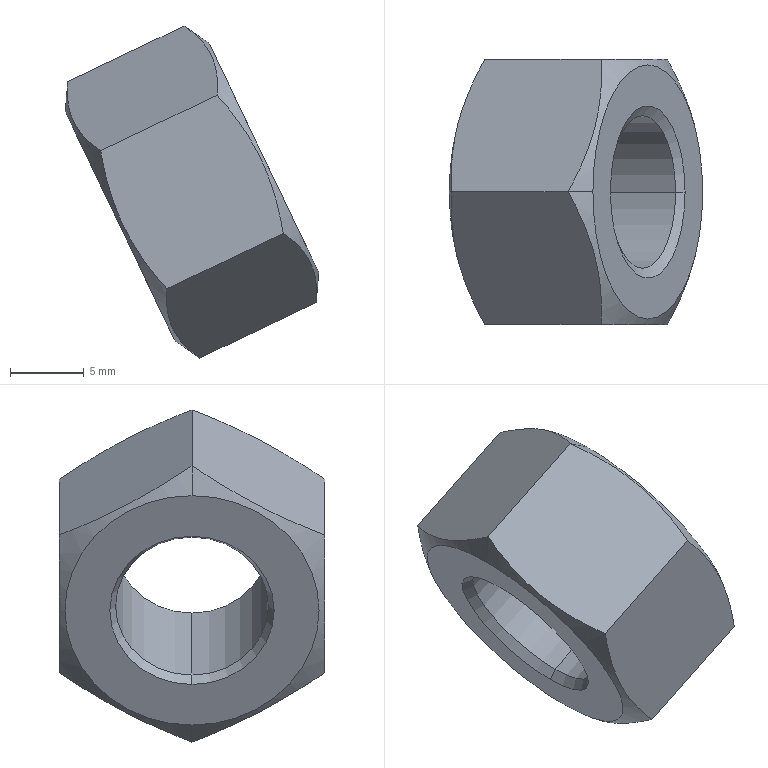Component | SolidWorks | hex nuts 1-fine pitch-grades ab gb-1 | 1 solid | 18 faces | box 17.19 x 18 x 22.53 mm | volume 2080 mm3 | cone 8 | plane 8 | cylinder 2 | commonest cylinder face diameters 10.376 x2
STEP:
#1=COLOUR_RGB('',0.7922,0.8196,0.9333);
#2=FILL_AREA_STYLE_COLOUR('',#1);
#3=FILL_AREA_STYLE('',(#2));
#4=SURFACE_STYLE_FILL_AREA(#3);
#5=SURFACE_SIDE_STYLE('',(#4));
#6=SURFACE_STYLE_USAGE(.BOTH.,#5);
#7=PRESENTATION_STYLE_ASSIGNMENT((#6));
#8=CARTESIAN_POINT('',(1.881,9.843,19.173));
#9=VERTEX_POINT('',#8);
#10=CARTESIAN_POINT('',(2.058,9.843,18.805));
#11=VERTEX_POINT('',#10);
#12=CARTESIAN_POINT('',(1.97,9.843,18.989));
#13=DIRECTION('',(0.902,-0.,0.4318));
#14=DIRECTION('',(-0.4318,-0.,0.902));
#15=AXIS2_PLACEMENT_3D('',#12,#13,#14);
#16=CIRCLE('',#15,0.2043);
#17=EDGE_CURVE('',#9,#11,#16,.T.);
#18=ORIENTED_EDGE('',*,*,#17,.F.);
#19=CARTESIAN_POINT('',(1.884,9.843,19.204));
#20=VERTEX_POINT('',#19);
#21=CARTESIAN_POINT('',(1.881,9.843,19.173));
#22=DIRECTION('',(0.07705,-0.,0.997));
#23=VECTOR('',#22,39.37);
#24=LINE('',#21,#23);
#25=EDGE_CURVE('',#9,#20,#24,.T.);
#26=ORIENTED_EDGE('',*,*,#25,.T.);
#27=CARTESIAN_POINT('',(2.083,9.843,18.788));
#28=VERTEX_POINT('',#27);
#29=CARTESIAN_POINT('',(1.983,9.843,18.996));
#30=DIRECTION('',(-0.902,0.,-0.4318));
#31=DIRECTION('',(-0.4318,-0.,0.902));
#32=AXIS2_PLACEMENT_3D('',#29,#30,#31);
#33=CIRCLE('',#32,0.2308);
#34=EDGE_CURVE('',#28,#20,#33,.T.);
#35=ORIENTED_EDGE('',*,*,#34,.F.);
#36=CARTESIAN_POINT('',(2.058,9.843,18.805));
#37=DIRECTION('',(0.8249,0.,-0.5652));
#38=VECTOR('',#37,39.37);
#39=LINE('',#36,#38);
#40=EDGE_CURVE('',#11,#28,#39,.T.);
#41=ORIENTED_EDGE('',*,*,#40,.F.);
#42=EDGE_LOOP('',(#18,#26,#35,#41));
#43=FACE_OUTER_BOUND('',#42,.T.);
#44=CARTESIAN_POINT('',(1.97,9.843,18.989));
#45=DIRECTION('',(0.902,-0.,0.4318));
#46=DIRECTION('',(0.4318,0.,-0.902));
#47=AXIS2_PLACEMENT_3D('',#44,#45,#46);
#48=CONICAL_SURFACE('',#47,0.2043,1.047);
#49=ADVANCED_FACE('',(#43),#48,.F.);
#50=CARTESIAN_POINT('',(1.712,9.843,18.64));
#51=VERTEX_POINT('',#50);
#52=CARTESIAN_POINT('',(1.536,9.843,19.008));
#53=VERTEX_POINT('',#52);
#54=CARTESIAN_POINT('',(1.624,9.843,18.824));
#55=DIRECTION('',(-0.902,0.,-0.4318));
#56=DIRECTION('',(-0.4318,-0.,0.902));
#57=AXIS2_PLACEMENT_3D('',#54,#55,#56);
#58=CIRCLE('',#57,0.2043);
#59=EDGE_CURVE('',#51,#53,#58,.T.);
#60=ORIENTED_EDGE('',*,*,#59,.F.);
#61=CARTESIAN_POINT('',(1.695,9.843,18.614));
#62=VERTEX_POINT('',#61);
#63=CARTESIAN_POINT('',(1.695,9.843,18.614));
#64=DIRECTION('',(-0.5652,0.,-0.8249));
#65=VECTOR('',#64,39.37);
#66=LINE('',#63,#65);
#67=EDGE_CURVE('',#51,#62,#66,.T.);
#68=ORIENTED_EDGE('',*,*,#67,.T.);
#69=CARTESIAN_POINT('',(1.505,9.843,19.01));
#70=VERTEX_POINT('',#69);
#71=CARTESIAN_POINT('',(1.6,9.843,18.812));
#72=DIRECTION('',(0.902,-0.,0.4318));
#73=DIRECTION('',(-0.4318,-0.,0.902));
#74=AXIS2_PLACEMENT_3D('',#71,#72,#73);
#75=CIRCLE('',#74,0.2196);
#76=EDGE_CURVE('',#70,#62,#75,.T.);
#77=ORIENTED_EDGE('',*,*,#76,.F.);
#78=CARTESIAN_POINT('',(1.505,9.843,19.01));
#79=DIRECTION('',(-0.997,-0.,0.07705));
#80=VECTOR('',#79,39.37);
#81=LINE('',#78,#80);
#82=EDGE_CURVE('',#53,#70,#81,.T.);
#83=ORIENTED_EDGE('',*,*,#82,.F.);
#84=EDGE_LOOP('',(#60,#68,#77,#83));
#85=FACE_OUTER_BOUND('',#84,.T.);
#86=CARTESIAN_POINT('',(1.6,9.843,18.812));
#87=DIRECTION('',(-0.902,0.,-0.4318));
#88=DIRECTION('',(-0.4318,-0.,0.902));
#89=AXIS2_PLACEMENT_3D('',#86,#87,#88);
#90=CONICAL_SURFACE('',#89,0.2196,0.5236);
#91=ADVANCED_FACE('',(#85),#90,.F.);
#92=CARTESIAN_POINT('',(1.837,9.843,19.302));
#93=VERTEX_POINT('',#92);
#94=CARTESIAN_POINT('',(2.13,9.843,18.69));
#95=VERTEX_POINT('',#94);
#96=CARTESIAN_POINT('',(1.983,9.843,18.996));
#97=DIRECTION('',(-0.902,0.,-0.4318));
#98=DIRECTION('',(-0.4318,-0.,0.902));
#99=AXIS2_PLACEMENT_3D('',#96,#97,#98);
#100=CIRCLE('',#99,0.3396);
#101=EDGE_CURVE('',#93,#95,#100,.T.);
#102=ORIENTED_EDGE('',*,*,#101,.T.);
#103=CARTESIAN_POINT('',(2.124,9.843,18.609));
#104=VERTEX_POINT('',#103);
#105=CARTESIAN_POINT('',(2.13,9.843,18.69));
#106=DIRECTION('',(-0.07705,0.,-0.997));
#107=VECTOR('',#106,39.37);
#108=LINE('',#105,#107);
#109=EDGE_CURVE('',#95,#104,#108,.T.);
#110=ORIENTED_EDGE('',*,*,#109,.T.);
#111=CARTESIAN_POINT('',(2.036,10.197,18.794));
#112=VERTEX_POINT('',#111);
#113=CARTESIAN_POINT('',(2.124,9.843,18.609));
#114=CARTESIAN_POINT('',(2.125,9.871,18.629));
#115=CARTESIAN_POINT('',(2.125,9.901,18.647));
#116=CARTESIAN_POINT('',(2.121,9.959,18.683));
#117=CARTESIAN_POINT('',(2.116,9.989,18.7));
#118=CARTESIAN_POINT('',(2.105,10.034,18.723));
#119=CARTESIAN_POINT('',(2.1,10.05,18.731));
#120=CARTESIAN_POINT('',(2.09,10.079,18.745));
#121=CARTESIAN_POINT('',(2.084,10.094,18.752));
#122=CARTESIAN_POINT('',(2.066,10.139,18.771));
#123=CARTESIAN_POINT('',(2.051,10.168,18.783));
#124=CARTESIAN_POINT('',(2.036,10.197,18.794));
#125=B_SPLINE_CURVE_WITH_KNOTS('',3,(#113,#114,#115,#116,#117,#118,#119,#120,#121,#122,#123,#124),.UNSPECIFIED.,.F.,.F.,(4,2,2,2,2,4),(0.00000024,0.002624,0.005248,0.00656,0.007872,0.0105),.UNSPECIFIED.);
#126=EDGE_CURVE('',#104,#112,#125,.T.);
#127=ORIENTED_EDGE('',*,*,#126,.T.);
#128=CARTESIAN_POINT('',(1.859,10.197,19.163));
#129=VERTEX_POINT('',#128);
#130=CARTESIAN_POINT('',(2.036,10.197,18.794));
#131=CARTESIAN_POINT('',(2.03,10.197,18.828));
#132=CARTESIAN_POINT('',(2.023,10.197,18.862));
#133=CARTESIAN_POINT('',(2.008,10.197,18.911));
#134=CARTESIAN_POINT('',(2.002,10.197,18.928));
#135=CARTESIAN_POINT('',(1.99,10.197,18.961));
#136=CARTESIAN_POINT('',(1.983,10.197,18.977));
#137=CARTESIAN_POINT('',(1.961,10.197,19.023));
#138=CARTESIAN_POINT('',(1.943,10.197,19.053));
#139=CARTESIAN_POINT('',(1.904,10.197,19.11));
#140=CARTESIAN_POINT('',(1.882,10.197,19.137));
#141=CARTESIAN_POINT('',(1.859,10.197,19.163));
#142=B_SPLINE_CURVE_WITH_KNOTS('',3,(#130,#131,#132,#133,#134,#135,#136,#137,#138,#139,#140,#141),.UNSPECIFIED.,.F.,.F.,(4,2,2,2,2,4),(0.003845,0.006467,0.007778,0.009089,0.01171,0.01433),.UNSPECIFIED.);
#143=EDGE_CURVE('',#112,#129,#142,.T.);
#144=ORIENTED_EDGE('',*,*,#143,.T.);
#145=CARTESIAN_POINT('',(1.771,9.843,19.348));
#146=VERTEX_POINT('',#145);
#147=CARTESIAN_POINT('',(1.859,10.197,19.163));
#148=CARTESIAN_POINT('',(1.86,10.168,19.182));
#149=CARTESIAN_POINT('',(1.86,10.139,19.201));
#150=CARTESIAN_POINT('',(1.856,10.08,19.236));
#151=CARTESIAN_POINT('',(1.851,10.05,19.253));
#152=CARTESIAN_POINT('',(1.84,10.005,19.277));
#153=CARTESIAN_POINT('',(1.835,9.99,19.284));
#154=CARTESIAN_POINT('',(1.825,9.96,19.299));
#155=CARTESIAN_POINT('',(1.819,9.945,19.305));
#156=CARTESIAN_POINT('',(1.801,9.901,19.325));
#157=CARTESIAN_POINT('',(1.786,9.871,19.337));
#158=CARTESIAN_POINT('',(1.771,9.843,19.348));
#159=B_SPLINE_CURVE_WITH_KNOTS('',3,(#147,#148,#149,#150,#151,#152,#153,#154,#155,#156,#157,#158),.UNSPECIFIED.,.F.,.F.,(4,2,2,2,2,4),(0.00000024,0.002624,0.005248,0.00656,0.007872,0.0105),.UNSPECIFIED.);
#160=EDGE_CURVE('',#129,#146,#159,.T.);
#161=ORIENTED_EDGE('',*,*,#160,.T.);
#162=CARTESIAN_POINT('',(1.837,9.843,19.302));
#163=DIRECTION('',(-0.8249,-0.,0.5652));
#164=VECTOR('',#163,39.37);
#165=LINE('',#162,#164);
#166=EDGE_CURVE('',#93,#146,#165,.T.);
#167=ORIENTED_EDGE('',*,*,#166,.F.);
#168=EDGE_LOOP('',(#102,#110,#127,#144,#161,#167));
#169=FACE_OUTER_BOUND('',#168,.T.);
#170=CARTESIAN_POINT('',(1.983,9.843,18.996));
#171=DIRECTION('',(-0.902,0.,-0.4318));
#172=DIRECTION('',(-0.4318,-0.,0.902));
#173=AXIS2_PLACEMENT_3D('',#170,#171,#172);
#174=CONICAL_SURFACE('',#173,0.3396,1.047);
#175=ADVANCED_FACE('',(#169),#174,.T.);
#176=CARTESIAN_POINT('',(1.453,9.843,19.119));
#177=VERTEX_POINT('',#176);
#178=CARTESIAN_POINT('',(1.747,9.843,18.506));
#179=VERTEX_POINT('',#178);
#180=CARTESIAN_POINT('',(1.6,9.843,18.812));
#181=DIRECTION('',(-0.902,0.,-0.4318));
#182=DIRECTION('',(-0.4318,-0.,0.902));
#183=AXIS2_PLACEMENT_3D('',#180,#181,#182);
#184=CIRCLE('',#183,0.3396);
#185=EDGE_CURVE('',#177,#179,#184,.T.);
#186=ORIENTED_EDGE('',*,*,#185,.F.);
#187=CARTESIAN_POINT('',(1.459,9.843,19.199));
#188=VERTEX_POINT('',#187);
#189=CARTESIAN_POINT('',(1.459,9.843,19.199));
#190=DIRECTION('',(0.07705,-0.,0.997));
#191=VECTOR('',#190,39.37);
#192=LINE('',#189,#191);
#193=EDGE_CURVE('',#177,#188,#192,.T.);
#194=ORIENTED_EDGE('',*,*,#193,.T.);
#195=CARTESIAN_POINT('',(1.548,10.197,19.014));
#196=VERTEX_POINT('',#195);
#197=CARTESIAN_POINT('',(1.459,9.843,19.199));
#198=CARTESIAN_POINT('',(1.458,9.871,19.179));
#199=CARTESIAN_POINT('',(1.458,9.901,19.161));
#200=CARTESIAN_POINT('',(1.463,9.959,19.125));
#201=CARTESIAN_POINT('',(1.468,9.989,19.109));
#202=CARTESIAN_POINT('',(1.479,10.034,19.085));
#203=CARTESIAN_POINT('',(1.483,10.05,19.078));
#204=CARTESIAN_POINT('',(1.493,10.079,19.063));
#205=CARTESIAN_POINT('',(1.499,10.094,19.056));
#206=CARTESIAN_POINT('',(1.517,10.139,19.037));
#207=CARTESIAN_POINT('',(1.532,10.168,19.025));
#208=CARTESIAN_POINT('',(1.548,10.197,19.014));
#209=B_SPLINE_CURVE_WITH_KNOTS('',3,(#197,#198,#199,#200,#201,#202,#203,#204,#205,#206,#207,#208),.UNSPECIFIED.,.F.,.F.,(4,2,2,2,2,4),(0.00000024,0.002624,0.005248,0.00656,0.007872,0.0105),.UNSPECIFIED.);
#210=EDGE_CURVE('',#188,#196,#209,.T.);
#211=ORIENTED_EDGE('',*,*,#210,.T.);
#212=CARTESIAN_POINT('',(1.724,10.197,18.645));
#213=VERTEX_POINT('',#212);
#214=CARTESIAN_POINT('',(1.548,10.197,19.014));
#215=CARTESIAN_POINT('',(1.554,10.197,18.98));
#216=CARTESIAN_POINT('',(1.561,10.197,18.946));
#217=CARTESIAN_POINT('',(1.581,10.197,18.879));
#218=CARTESIAN_POINT('',(1.593,10.197,18.847));
#219=CARTESIAN_POINT('',(1.615,10.197,18.8));
#220=CARTESIAN_POINT('',(1.623,10.197,18.785));
#221=CARTESIAN_POINT('',(1.641,10.197,18.755));
#222=CARTESIAN_POINT('',(1.65,10.197,18.74));
#223=CARTESIAN_POINT('',(1.68,10.197,18.698));
#224=CARTESIAN_POINT('',(1.702,10.197,18.671));
#225=CARTESIAN_POINT('',(1.724,10.197,18.645));
#226=B_SPLINE_CURVE_WITH_KNOTS('',3,(#214,#215,#216,#217,#218,#219,#220,#221,#222,#223,#224,#225),.UNSPECIFIED.,.F.,.F.,(4,2,2,2,2,4),(0.009237,0.01187,0.0145,0.01581,0.01712,0.01975),.UNSPECIFIED.);
#227=EDGE_CURVE('',#196,#213,#226,.T.);
#228=ORIENTED_EDGE('',*,*,#227,.T.);
#229=CARTESIAN_POINT('',(1.813,9.843,18.461));
#230=VERTEX_POINT('',#229);
#231=CARTESIAN_POINT('',(1.724,10.197,18.645));
#232=CARTESIAN_POINT('',(1.723,10.168,18.626));
#233=CARTESIAN_POINT('',(1.723,10.139,18.607));
#234=CARTESIAN_POINT('',(1.728,10.08,18.572));
#235=CARTESIAN_POINT('',(1.733,10.05,18.555));
#236=CARTESIAN_POINT('',(1.744,10.005,18.532));
#237=CARTESIAN_POINT('',(1.748,9.99,18.524));
#238=CARTESIAN_POINT('',(1.758,9.96,18.51));
#239=CARTESIAN_POINT('',(1.764,9.945,18.503));
#240=CARTESIAN_POINT('',(1.782,9.901,18.483));
#241=CARTESIAN_POINT('',(1.797,9.871,18.472));
#242=CARTESIAN_POINT('',(1.813,9.843,18.461));
#243=B_SPLINE_CURVE_WITH_KNOTS('',3,(#231,#232,#233,#234,#235,#236,#237,#238,#239,#240,#241,#242),.UNSPECIFIED.,.F.,.F.,(4,2,2,2,2,4),(0.00000024,0.002624,0.005248,0.00656,0.007872,0.0105),.UNSPECIFIED.);
#244=EDGE_CURVE('',#213,#230,#243,.T.);
#245=ORIENTED_EDGE('',*,*,#244,.T.);
#246=CARTESIAN_POINT('',(1.813,9.843,18.461));
#247=DIRECTION('',(0.8249,0.,-0.5652));
#248=VECTOR('',#247,39.37);
#249=LINE('',#246,#248);
#250=EDGE_CURVE('',#179,#230,#249,.T.);
#251=ORIENTED_EDGE('',*,*,#250,.F.);
#252=EDGE_LOOP('',(#186,#194,#211,#228,#245,#251));
#253=FACE_OUTER_BOUND('',#252,.T.);
#254=CARTESIAN_POINT('',(1.636,9.843,18.83));
#255=DIRECTION('',(0.902,-0.,0.4318));
#256=DIRECTION('',(0.4318,0.,-0.902));
#257=AXIS2_PLACEMENT_3D('',#254,#255,#256);
#258=CONICAL_SURFACE('',#257,0.4091,1.047);
#259=ADVANCED_FACE('',(#253),#258,.T.);
#260=ORIENTED_EDGE('',*,*,#59,.T.);
#261=CARTESIAN_POINT('',(1.512,9.843,18.997));
#262=DIRECTION('',(0.902,-0.,0.4318));
#263=VECTOR('',#262,39.37);
#264=LINE('',#261,#263);
#265=EDGE_CURVE('',#53,#9,#264,.T.);
#266=ORIENTED_EDGE('',*,*,#265,.T.);
#267=ORIENTED_EDGE('',*,*,#17,.T.);
#268=CARTESIAN_POINT('',(1.688,9.843,18.628));
#269=DIRECTION('',(0.902,-0.,0.4318));
#270=VECTOR('',#269,39.37);
#271=LINE('',#268,#270);
#272=EDGE_CURVE('',#51,#11,#271,.T.);
#273=ORIENTED_EDGE('',*,*,#272,.F.);
#274=EDGE_LOOP('',(#260,#266,#267,#273));
#275=FACE_OUTER_BOUND('',#274,.T.);
#276=CARTESIAN_POINT('',(1.6,9.843,18.812));
#277=DIRECTION('',(0.902,-0.,0.4318));
#278=DIRECTION('',(0.4318,0.,-0.902));
#279=AXIS2_PLACEMENT_3D('',#276,#277,#278);
#280=CYLINDRICAL_SURFACE('',#279,0.2043);
#281=ADVANCED_FACE('',(#275),#280,.F.);
#282=CARTESIAN_POINT('',(1.859,9.488,19.163));
#283=VERTEX_POINT('',#282);
#284=CARTESIAN_POINT('',(2.036,9.488,18.794));
#285=VERTEX_POINT('',#284);
#286=CARTESIAN_POINT('',(1.859,9.488,19.163));
#287=CARTESIAN_POINT('',(1.882,9.488,19.137));
#288=CARTESIAN_POINT('',(1.904,9.488,19.11));
#289=CARTESIAN_POINT('',(1.943,9.488,19.053));
#290=CARTESIAN_POINT('',(1.961,9.488,19.023));
#291=CARTESIAN_POINT('',(1.983,9.488,18.977));
#292=CARTESIAN_POINT('',(1.99,9.488,18.961));
#293=CARTESIAN_POINT('',(2.002,9.488,18.928));
#294=CARTESIAN_POINT('',(2.008,9.488,18.911));
#295=CARTESIAN_POINT('',(2.023,9.488,18.862));
#296=CARTESIAN_POINT('',(2.03,9.488,18.828));
#297=CARTESIAN_POINT('',(2.036,9.488,18.794));
#298=B_SPLINE_CURVE_WITH_KNOTS('',3,(#286,#287,#288,#289,#290,#291,#292,#293,#294,#295,#296,#297),.UNSPECIFIED.,.F.,.F.,(4,2,2,2,2,4),(0.009237,0.01187,0.0145,0.01581,0.01712,0.01975),.UNSPECIFIED.);
#299=EDGE_CURVE('',#283,#285,#298,.T.);
#300=ORIENTED_EDGE('',*,*,#299,.F.);
#301=CARTESIAN_POINT('',(1.548,9.488,19.014));
#302=VERTEX_POINT('',#301);
#303=CARTESIAN_POINT('',(1.512,9.488,18.997));
#304=DIRECTION('',(0.902,-0.,0.4318));
#305=VECTOR('',#304,39.37);
#306=LINE('',#303,#305);
#307=EDGE_CURVE('',#302,#283,#306,.T.);
#308=ORIENTED_EDGE('',*,*,#307,.F.);
#309=CARTESIAN_POINT('',(1.724,9.488,18.645));
#310=VERTEX_POINT('',#309);
#311=CARTESIAN_POINT('',(1.724,9.488,18.645));
#312=CARTESIAN_POINT('',(1.702,9.488,18.671));
#313=CARTESIAN_POINT('',(1.68,9.488,18.698));
#314=CARTESIAN_POINT('',(1.65,9.488,18.74));
#315=CARTESIAN_POINT('',(1.641,9.488,18.755));
#316=CARTESIAN_POINT('',(1.623,9.488,18.785));
#317=CARTESIAN_POINT('',(1.615,9.488,18.8));
#318=CARTESIAN_POINT('',(1.593,9.488,18.847));
#319=CARTESIAN_POINT('',(1.581,9.488,18.879));
#320=CARTESIAN_POINT('',(1.561,9.488,18.946));
#321=CARTESIAN_POINT('',(1.554,9.488,18.98));
#322=CARTESIAN_POINT('',(1.548,9.488,19.014));
#323=B_SPLINE_CURVE_WITH_KNOTS('',3,(#311,#312,#313,#314,#315,#316,#317,#318,#319,#320,#321,#322),.UNSPECIFIED.,.F.,.F.,(4,2,2,2,2,4),(0.003845,0.006467,0.007778,0.009089,0.01171,0.01433),.UNSPECIFIED.);
#324=EDGE_CURVE('',#310,#302,#323,.T.);
#325=ORIENTED_EDGE('',*,*,#324,.F.);
#326=CARTESIAN_POINT('',(1.688,9.488,18.628));
#327=DIRECTION('',(0.902,-0.,0.4318));
#328=VECTOR('',#327,39.37);
#329=LINE('',#326,#328);
#330=EDGE_CURVE('',#310,#285,#329,.T.);
#331=ORIENTED_EDGE('',*,*,#330,.T.);
#332=EDGE_LOOP('',(#300,#308,#325,#331));
#333=FACE_OUTER_BOUND('',#332,.T.);
#334=CARTESIAN_POINT('',(1.512,9.488,18.997));
#335=DIRECTION('',(0.,-1.,-0.));
#336=DIRECTION('',(0.4318,0.,-0.902));
#337=AXIS2_PLACEMENT_3D('',#334,#335,#336);
#338=PLANE('',#337);
#339=ADVANCED_FACE('',(#333),#338,.T.);
#340=CARTESIAN_POINT('',(1.771,9.843,19.348));
#341=CARTESIAN_POINT('',(1.786,9.814,19.337));
#342=CARTESIAN_POINT('',(1.801,9.784,19.325));
#343=CARTESIAN_POINT('',(1.825,9.726,19.299));
#344=CARTESIAN_POINT('',(1.836,9.696,19.285));
#345=CARTESIAN_POINT('',(1.847,9.651,19.261));
#346=CARTESIAN_POINT('',(1.85,9.635,19.253));
#347=CARTESIAN_POINT('',(1.855,9.606,19.236));
#348=CARTESIAN_POINT('',(1.857,9.591,19.228));
#349=CARTESIAN_POINT('',(1.86,9.546,19.201));
#350=CARTESIAN_POINT('',(1.86,9.517,19.182));
#351=CARTESIAN_POINT('',(1.859,9.488,19.163));
#352=B_SPLINE_CURVE_WITH_KNOTS('',3,(#340,#341,#342,#343,#344,#345,#346,#347,#348,#349,#350,#351),.UNSPECIFIED.,.F.,.F.,(4,2,2,2,2,4),(0.00000024,0.002624,0.005248,0.00656,0.007872,0.0105),.UNSPECIFIED.);
#353=EDGE_CURVE('',#146,#283,#352,.T.);
#354=ORIENTED_EDGE('',*,*,#353,.F.);
#355=CARTESIAN_POINT('',(1.423,9.843,19.181));
#356=DIRECTION('',(0.902,-0.,0.4318));
#357=VECTOR('',#356,39.37);
#358=LINE('',#355,#357);
#359=EDGE_CURVE('',#188,#146,#358,.T.);
#360=ORIENTED_EDGE('',*,*,#359,.F.);
#361=CARTESIAN_POINT('',(1.548,9.488,19.014));
#362=CARTESIAN_POINT('',(1.532,9.517,19.025));
#363=CARTESIAN_POINT('',(1.517,9.546,19.037));
#364=CARTESIAN_POINT('',(1.493,9.605,19.063));
#365=CARTESIAN_POINT('',(1.483,9.635,19.077));
#366=CARTESIAN_POINT('',(1.471,9.68,19.1));
#367=CARTESIAN_POINT('',(1.468,9.695,19.109));
#368=CARTESIAN_POINT('',(1.463,9.725,19.125));
#369=CARTESIAN_POINT('',(1.462,9.74,19.134));
#370=CARTESIAN_POINT('',(1.458,9.784,19.161));
#371=CARTESIAN_POINT('',(1.458,9.814,19.179));
#372=CARTESIAN_POINT('',(1.459,9.843,19.199));
#373=B_SPLINE_CURVE_WITH_KNOTS('',3,(#361,#362,#363,#364,#365,#366,#367,#368,#369,#370,#371,#372),.UNSPECIFIED.,.F.,.F.,(4,2,2,2,2,4),(0.00000024,0.002624,0.005248,0.00656,0.007872,0.0105),.UNSPECIFIED.);
#374=EDGE_CURVE('',#302,#188,#373,.T.);
#375=ORIENTED_EDGE('',*,*,#374,.F.);
#376=ORIENTED_EDGE('',*,*,#307,.T.);
#377=EDGE_LOOP('',(#354,#360,#375,#376));
#378=FACE_OUTER_BOUND('',#377,.T.);
#379=CARTESIAN_POINT('',(1.423,9.843,19.181));
#380=DIRECTION('',(-0.3739,-0.5,0.7811));
#381=DIRECTION('',(0.2159,-0.866,-0.451));
#382=AXIS2_PLACEMENT_3D('',#379,#380,#381);
#383=PLANE('',#382);
#384=ADVANCED_FACE('',(#378),#383,.T.);
#385=ORIENTED_EDGE('',*,*,#160,.F.);
#386=CARTESIAN_POINT('',(1.512,10.197,18.997));
#387=DIRECTION('',(0.902,-0.,0.4318));
#388=VECTOR('',#387,39.37);
#389=LINE('',#386,#388);
#390=EDGE_CURVE('',#196,#129,#389,.T.);
#391=ORIENTED_EDGE('',*,*,#390,.F.);
#392=ORIENTED_EDGE('',*,*,#210,.F.);
#393=ORIENTED_EDGE('',*,*,#359,.T.);
#394=EDGE_LOOP('',(#385,#391,#392,#393));
#395=FACE_OUTER_BOUND('',#394,.T.);
#396=CARTESIAN_POINT('',(1.512,10.197,18.997));
#397=DIRECTION('',(-0.3739,0.5,0.7811));
#398=DIRECTION('',(-0.2159,-0.866,0.451));
#399=AXIS2_PLACEMENT_3D('',#396,#397,#398);
#400=PLANE('',#399);
#401=ADVANCED_FACE('',(#395),#400,.T.);
#402=ORIENTED_EDGE('',*,*,#143,.F.);
#403=CARTESIAN_POINT('',(1.688,10.197,18.628));
#404=DIRECTION('',(0.902,-0.,0.4318));
#405=VECTOR('',#404,39.37);
#406=LINE('',#403,#405);
#407=EDGE_CURVE('',#213,#112,#406,.T.);
#408=ORIENTED_EDGE('',*,*,#407,.F.);
#409=ORIENTED_EDGE('',*,*,#227,.F.);
#410=ORIENTED_EDGE('',*,*,#390,.T.);
#411=EDGE_LOOP('',(#402,#408,#409,#410));
#412=FACE_OUTER_BOUND('',#411,.T.);
#413=CARTESIAN_POINT('',(1.688,10.197,18.628));
#414=DIRECTION('',(-0.,1.,0.));
#415=DIRECTION('',(0.902,-0.,0.4318));
#416=AXIS2_PLACEMENT_3D('',#413,#414,#415);
#417=PLANE('',#416);
#418=ADVANCED_FACE('',(#412),#417,.T.);
#419=ORIENTED_EDGE('',*,*,#126,.F.);
#420=CARTESIAN_POINT('',(1.777,9.843,18.443));
#421=DIRECTION('',(0.902,-0.,0.4318));
#422=VECTOR('',#421,39.37);
#423=LINE('',#420,#422);
#424=EDGE_CURVE('',#230,#104,#423,.T.);
#425=ORIENTED_EDGE('',*,*,#424,.F.);
#426=ORIENTED_EDGE('',*,*,#244,.F.);
#427=ORIENTED_EDGE('',*,*,#407,.T.);
#428=EDGE_LOOP('',(#419,#425,#426,#427));
#429=FACE_OUTER_BOUND('',#428,.T.);
#430=CARTESIAN_POINT('',(1.777,9.843,18.443));
#431=DIRECTION('',(0.3739,0.5,-0.7811));
#432=DIRECTION('',(-0.2159,0.866,0.451));
#433=AXIS2_PLACEMENT_3D('',#430,#431,#432);
#434=PLANE('',#433);
#435=ADVANCED_FACE('',(#429),#434,.T.);
#436=CARTESIAN_POINT('',(2.036,9.488,18.794));
#437=CARTESIAN_POINT('',(2.051,9.517,18.783));
#438=CARTESIAN_POINT('',(2.066,9.546,18.771));
#439=CARTESIAN_POINT('',(2.09,9.605,18.745));
#440=CARTESIAN_POINT('',(2.101,9.635,18.731));
#441=CARTESIAN_POINT('',(2.112,9.68,18.708));
#442=CARTESIAN_POINT('',(2.115,9.695,18.7));
#443=CARTESIAN_POINT('',(2.12,9.725,18.683));
#444=CARTESIAN_POINT('',(2.122,9.74,18.674));
#445=CARTESIAN_POINT('',(2.125,9.784,18.647));
#446=CARTESIAN_POINT('',(2.125,9.814,18.629));
#447=CARTESIAN_POINT('',(2.124,9.843,18.609));
#448=B_SPLINE_CURVE_WITH_KNOTS('',3,(#436,#437,#438,#439,#440,#441,#442,#443,#444,#445,#446,#447),.UNSPECIFIED.,.F.,.F.,(4,2,2,2,2,4),(0.00000024,0.002624,0.005248,0.00656,0.007872,0.0105),.UNSPECIFIED.);
#449=EDGE_CURVE('',#285,#104,#448,.T.);
#450=ORIENTED_EDGE('',*,*,#449,.F.);
#451=ORIENTED_EDGE('',*,*,#330,.F.);
#452=CARTESIAN_POINT('',(1.813,9.843,18.461));
#453=CARTESIAN_POINT('',(1.797,9.814,18.471));
#454=CARTESIAN_POINT('',(1.782,9.784,18.483));
#455=CARTESIAN_POINT('',(1.758,9.726,18.509));
#456=CARTESIAN_POINT('',(1.748,9.696,18.523));
#457=CARTESIAN_POINT('',(1.736,9.651,18.547));
#458=CARTESIAN_POINT('',(1.733,9.635,18.555));
#459=CARTESIAN_POINT('',(1.728,9.606,18.572));
#460=CARTESIAN_POINT('',(1.727,9.591,18.581));
#461=CARTESIAN_POINT('',(1.723,9.546,18.607));
#462=CARTESIAN_POINT('',(1.723,9.517,18.626));
#463=CARTESIAN_POINT('',(1.724,9.488,18.645));
#464=B_SPLINE_CURVE_WITH_KNOTS('',3,(#452,#453,#454,#455,#456,#457,#458,#459,#460,#461,#462,#463),.UNSPECIFIED.,.F.,.F.,(4,2,2,2,2,4),(0.00000024,0.002624,0.005248,0.00656,0.007872,0.0105),.UNSPECIFIED.);
#465=EDGE_CURVE('',#230,#310,#464,.T.);
#466=ORIENTED_EDGE('',*,*,#465,.F.);
#467=ORIENTED_EDGE('',*,*,#424,.T.);
#468=EDGE_LOOP('',(#450,#451,#466,#467));
#469=FACE_OUTER_BOUND('',#468,.T.);
#470=CARTESIAN_POINT('',(1.688,9.488,18.628));
#471=DIRECTION('',(0.3739,-0.5,-0.7811));
#472=DIRECTION('',(0.2159,0.866,-0.451));
#473=AXIS2_PLACEMENT_3D('',#470,#471,#472);
#474=PLANE('',#473);
#475=ADVANCED_FACE('',(#469),#474,.T.);
#476=ORIENTED_EDGE('',*,*,#76,.T.);
#477=CARTESIAN_POINT('',(1.6,9.843,18.812));
#478=DIRECTION('',(0.902,-0.,0.4318));
#479=DIRECTION('',(-0.4318,-0.,0.902));
#480=AXIS2_PLACEMENT_3D('',#477,#478,#479);
#481=CIRCLE('',#480,0.2196);
#482=EDGE_CURVE('',#62,#70,#481,.T.);
#483=ORIENTED_EDGE('',*,*,#482,.T.);
#484=EDGE_LOOP('',(#476,#483));
#485=FACE_BOUND('',#484,.T.);
#486=CARTESIAN_POINT('',(1.6,9.843,18.812));
#487=DIRECTION('',(-0.902,0.,-0.4318));
#488=DIRECTION('',(-0.4318,-0.,0.902));
#489=AXIS2_PLACEMENT_3D('',#486,#487,#488);
#490=CIRCLE('',#489,0.3396);
#491=EDGE_CURVE('',#179,#177,#490,.T.);
#492=ORIENTED_EDGE('',*,*,#491,.T.);
#493=ORIENTED_EDGE('',*,*,#185,.T.);
#494=EDGE_LOOP('',(#492,#493));
#495=FACE_OUTER_BOUND('',#494,.T.);
#496=CARTESIAN_POINT('',(1.512,9.488,18.997));
#497=DIRECTION('',(-0.902,0.,-0.4318));
#498=DIRECTION('',(-0.4318,-0.,0.902));
#499=AXIS2_PLACEMENT_3D('',#496,#497,#498);
#500=PLANE('',#499);
#501=ADVANCED_FACE('',(#485,#495),#500,.T.);
#502=ORIENTED_EDGE('',*,*,#34,.T.);
#503=CARTESIAN_POINT('',(1.983,9.843,18.996));
#504=DIRECTION('',(-0.902,0.,-0.4318));
#505=DIRECTION('',(-0.4318,-0.,0.902));
#506=AXIS2_PLACEMENT_3D('',#503,#504,#505);
#507=CIRCLE('',#506,0.2308);
#508=EDGE_CURVE('',#20,#28,#507,.T.);
#509=ORIENTED_EDGE('',*,*,#508,.T.);
#510=EDGE_LOOP('',(#502,#509));
#511=FACE_BOUND('',#510,.T.);
#512=ORIENTED_EDGE('',*,*,#101,.F.);
#513=CARTESIAN_POINT('',(1.983,9.843,18.996));
#514=DIRECTION('',(-0.902,0.,-0.4318));
#515=DIRECTION('',(-0.4318,-0.,0.902));
#516=AXIS2_PLACEMENT_3D('',#513,#514,#515);
#517=CIRCLE('',#516,0.3396);
#518=EDGE_CURVE('',#95,#93,#517,.T.);
#519=ORIENTED_EDGE('',*,*,#518,.F.);
#520=EDGE_LOOP('',(#512,#519));
#521=FACE_OUTER_BOUND('',#520,.T.);
#522=CARTESIAN_POINT('',(1.895,9.488,19.18));
#523=DIRECTION('',(-0.902,0.,-0.4318));
#524=DIRECTION('',(-0.4318,-0.,0.902));
#525=AXIS2_PLACEMENT_3D('',#522,#523,#524);
#526=PLANE('',#525);
#527=ADVANCED_FACE('',(#511,#521),#526,.F.);
#528=ORIENTED_EDGE('',*,*,#265,.F.);
#529=CARTESIAN_POINT('',(1.624,9.843,18.824));
#530=DIRECTION('',(-0.902,0.,-0.4318));
#531=DIRECTION('',(-0.4318,-0.,0.902));
#532=AXIS2_PLACEMENT_3D('',#529,#530,#531);
#533=CIRCLE('',#532,0.2043);
#534=EDGE_CURVE('',#53,#51,#533,.T.);
#535=ORIENTED_EDGE('',*,*,#534,.T.);
#536=ORIENTED_EDGE('',*,*,#272,.T.);
#537=CARTESIAN_POINT('',(1.97,9.843,18.989));
#538=DIRECTION('',(0.902,-0.,0.4318));
#539=DIRECTION('',(-0.4318,-0.,0.902));
#540=AXIS2_PLACEMENT_3D('',#537,#538,#539);
#541=CIRCLE('',#540,0.2043);
#542=EDGE_CURVE('',#11,#9,#541,.T.);
#543=ORIENTED_EDGE('',*,*,#542,.T.);
#544=EDGE_LOOP('',(#528,#535,#536,#543));
#545=FACE_OUTER_BOUND('',#544,.T.);
#546=CARTESIAN_POINT('',(1.6,9.843,18.812));
#547=DIRECTION('',(0.902,-0.,0.4318));
#548=DIRECTION('',(0.4318,0.,-0.902));
#549=AXIS2_PLACEMENT_3D('',#546,#547,#548);
#550=CYLINDRICAL_SURFACE('',#549,0.2043);
#551=ADVANCED_FACE('',(#545),#550,.F.);
#552=ORIENTED_EDGE('',*,*,#193,.F.);
#553=ORIENTED_EDGE('',*,*,#491,.F.);
#554=ORIENTED_EDGE('',*,*,#250,.T.);
#555=ORIENTED_EDGE('',*,*,#465,.T.);
#556=ORIENTED_EDGE('',*,*,#324,.T.);
#557=ORIENTED_EDGE('',*,*,#374,.T.);
#558=EDGE_LOOP('',(#552,#553,#554,#555,#556,#557));
#559=FACE_OUTER_BOUND('',#558,.T.);
#560=CARTESIAN_POINT('',(1.636,9.843,18.83));
#561=DIRECTION('',(0.902,-0.,0.4318));
#562=DIRECTION('',(0.4318,0.,-0.902));
#563=AXIS2_PLACEMENT_3D('',#560,#561,#562);
#564=CONICAL_SURFACE('',#563,0.4091,1.047);
#565=ADVANCED_FACE('',(#559),#564,.T.);
#566=ORIENTED_EDGE('',*,*,#109,.F.);
#567=ORIENTED_EDGE('',*,*,#518,.T.);
#568=ORIENTED_EDGE('',*,*,#166,.T.);
#569=ORIENTED_EDGE('',*,*,#353,.T.);
#570=ORIENTED_EDGE('',*,*,#299,.T.);
#571=ORIENTED_EDGE('',*,*,#449,.T.);
#572=EDGE_LOOP('',(#566,#567,#568,#569,#570,#571));
#573=FACE_OUTER_BOUND('',#572,.T.);
#574=CARTESIAN_POINT('',(1.983,9.843,18.996));
#575=DIRECTION('',(-0.902,0.,-0.4318));
#576=DIRECTION('',(-0.4318,-0.,0.902));
#577=AXIS2_PLACEMENT_3D('',#574,#575,#576);
#578=CONICAL_SURFACE('',#577,0.3396,1.047);
#579=ADVANCED_FACE('',(#573),#578,.T.);
#580=ORIENTED_EDGE('',*,*,#67,.F.);
#581=ORIENTED_EDGE('',*,*,#534,.F.);
#582=ORIENTED_EDGE('',*,*,#82,.T.);
#583=ORIENTED_EDGE('',*,*,#482,.F.);
#584=EDGE_LOOP('',(#580,#581,#582,#583));
#585=FACE_OUTER_BOUND('',#584,.T.);
#586=CARTESIAN_POINT('',(1.6,9.843,18.812));
#587=DIRECTION('',(-0.902,0.,-0.4318));
#588=DIRECTION('',(-0.4318,-0.,0.902));
#589=AXIS2_PLACEMENT_3D('',#586,#587,#588);
#590=CONICAL_SURFACE('',#589,0.2196,0.5236);
#591=ADVANCED_FACE('',(#585),#590,.F.);
#592=ORIENTED_EDGE('',*,*,#25,.F.);
#593=ORIENTED_EDGE('',*,*,#542,.F.);
#594=ORIENTED_EDGE('',*,*,#40,.T.);
#595=ORIENTED_EDGE('',*,*,#508,.F.);
#596=EDGE_LOOP('',(#592,#593,#594,#595));
#597=FACE_OUTER_BOUND('',#596,.T.);
#598=CARTESIAN_POINT('',(1.97,9.843,18.989));
#599=DIRECTION('',(0.902,-0.,0.4318));
#600=DIRECTION('',(0.4318,0.,-0.902));
#601=AXIS2_PLACEMENT_3D('',#598,#599,#600);
#602=CONICAL_SURFACE('',#601,0.2043,1.047);
#603=ADVANCED_FACE('',(#597),#602,.F.);
#604=CLOSED_SHELL('',(#49,#91,#175,#259,#281,#339,#384,#401,#418,#435,#475,#501,#527,#551,#565,#579,#591,#603));
#605=MANIFOLD_SOLID_BREP('',#604);
#606=STYLED_ITEM('',(#7),#605);
#607=(LENGTH_UNIT()NAMED_UNIT(*)SI_UNIT($,.METRE.));
#608=LENGTH_MEASURE_WITH_UNIT(LENGTH_MEASURE(0.0254),#607);
#609=DIMENSIONAL_EXPONENTS(1.,0.,0.,0.,0.,0.,0.);
#610=(CONVERSION_BASED_UNIT('',#608)LENGTH_UNIT()NAMED_UNIT(#609));
#611=UNCERTAINTY_MEASURE_WITH_UNIT(LENGTH_MEASURE(0.00001),#610,'','');
#612=(NAMED_UNIT(*)PLANE_ANGLE_UNIT()SI_UNIT($,.RADIAN.));
#613=(NAMED_UNIT(*)SI_UNIT($,.STERADIAN.)SOLID_ANGLE_UNIT());
#614=(GEOMETRIC_REPRESENTATION_CONTEXT(3)GLOBAL_UNCERTAINTY_ASSIGNED_CONTEXT((#611))GLOBAL_UNIT_ASSIGNED_CONTEXT((#610,#612,#613))REPRESENTATION_CONTEXT('',''));
#615=MECHANICAL_DESIGN_GEOMETRIC_PRESENTATION_REPRESENTATION('',(#606),#614);
#616=CARTESIAN_POINT('',(0.,0.,0.));
#617=DIRECTION('',(0.,0.,1.));
#618=DIRECTION('',(1.,0.,0.));
#619=AXIS2_PLACEMENT_3D('',#616,#617,#618);
#620=(LENGTH_UNIT()NAMED_UNIT(*)SI_UNIT($,.METRE.));
#621=LENGTH_MEASURE_WITH_UNIT(LENGTH_MEASURE(0.0254),#620);
#622=DIMENSIONAL_EXPONENTS(1.,0.,0.,0.,0.,0.,0.);
#623=(CONVERSION_BASED_UNIT('',#621)LENGTH_UNIT()NAMED_UNIT(#622));
#624=UNCERTAINTY_MEASURE_WITH_UNIT(LENGTH_MEASURE(0.00001),#623,'','');
#625=(NAMED_UNIT(*)PLANE_ANGLE_UNIT()SI_UNIT($,.RADIAN.));
#626=(NAMED_UNIT(*)SI_UNIT($,.STERADIAN.)SOLID_ANGLE_UNIT());
#627=(GEOMETRIC_REPRESENTATION_CONTEXT(3)GLOBAL_UNCERTAINTY_ASSIGNED_CONTEXT((#624))GLOBAL_UNIT_ASSIGNED_CONTEXT((#623,#625,#626))REPRESENTATION_CONTEXT('',''));
#628=ADVANCED_BREP_SHAPE_REPRESENTATION('',(#605,#619),#627);
#629=PRESENTATION_LAYER_ASSIGNMENT('','',(#606));